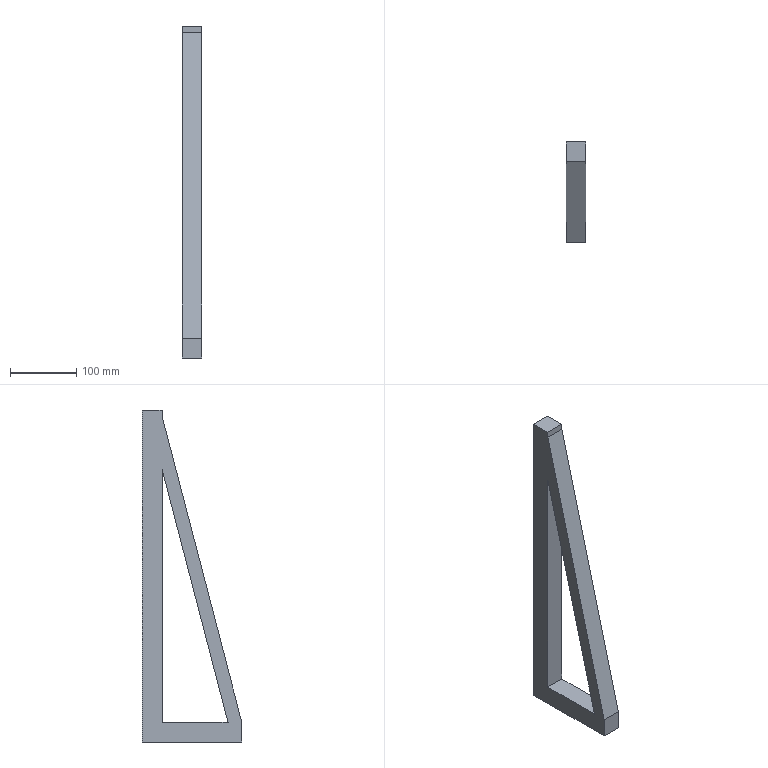Component | SolidWorks | LiftingArm122-1 | 1 solid | 11 faces | box 30 x 150 x 500 mm | volume 818896 mm3 | plane 11
build123d program:
from build123d import *

# Parameters (mm, degrees)
BOSS_EXTRUDE1_DEPTH = 30


with BuildPart() as part:
    # Sketch1 → Boss-Extrude1 (new body)
    with BuildSketch(Plane.XY):
        Polygon((0, 0), (500, 0), (500, -30), (490.421, -30), (30, -150), (0, -150), align=None)
        Polygon((30, -30), (411.12, -30), (30, -129.332), align=None, mode=Mode.SUBTRACT)
    extrude(amount=BOSS_EXTRUDE1_DEPTH)


solid = part.part

# Placed as in the assembly
solid = solid.moved(Location((-219.479, 25.652, 889.07), (0, -90, 0)))
STEP:
#1=COLOUR_RGB('',0.7922,0.8196,0.9333);
#2=FILL_AREA_STYLE_COLOUR('',#1);
#3=FILL_AREA_STYLE('',(#2));
#4=SURFACE_STYLE_FILL_AREA(#3);
#5=SURFACE_SIDE_STYLE('',(#4));
#6=SURFACE_STYLE_USAGE(.BOTH.,#5);
#7=PRESENTATION_STYLE_ASSIGNMENT((#6));
#8=CARTESIAN_POINT('',(-9.822,1.01,35.003));
#9=VERTEX_POINT('',#8);
#10=CARTESIAN_POINT('',(-9.822,-4.896,35.003));
#11=VERTEX_POINT('',#10);
#12=CARTESIAN_POINT('',(-9.822,-4.896,35.003));
#13=DIRECTION('',(0.,-1.,0.));
#14=VECTOR('',#13,39.37);
#15=LINE('',#12,#14);
#16=EDGE_CURVE('',#9,#11,#15,.T.);
#17=ORIENTED_EDGE('',*,*,#16,.T.);
#18=CARTESIAN_POINT('',(-9.822,-4.896,36.184));
#19=VERTEX_POINT('',#18);
#20=CARTESIAN_POINT('',(-9.822,-4.896,36.184));
#21=DIRECTION('',(0.,0.,1.));
#22=VECTOR('',#21,39.37);
#23=LINE('',#20,#22);
#24=EDGE_CURVE('',#11,#19,#23,.T.);
#25=ORIENTED_EDGE('',*,*,#24,.T.);
#26=CARTESIAN_POINT('',(-9.822,-0.1712,54.311));
#27=VERTEX_POINT('',#26);
#28=CARTESIAN_POINT('',(-9.822,-4.896,36.184));
#29=DIRECTION('',(0.,0.2522,0.9677));
#30=VECTOR('',#29,39.37);
#31=LINE('',#28,#30);
#32=EDGE_CURVE('',#19,#27,#31,.T.);
#33=ORIENTED_EDGE('',*,*,#32,.T.);
#34=CARTESIAN_POINT('',(-9.822,-0.1712,54.688));
#35=VERTEX_POINT('',#34);
#36=CARTESIAN_POINT('',(-9.822,-0.1712,54.311));
#37=DIRECTION('',(0.,0.,1.));
#38=VECTOR('',#37,39.37);
#39=LINE('',#36,#38);
#40=EDGE_CURVE('',#27,#35,#39,.T.);
#41=ORIENTED_EDGE('',*,*,#40,.T.);
#42=CARTESIAN_POINT('',(-9.822,1.01,54.688));
#43=VERTEX_POINT('',#42);
#44=CARTESIAN_POINT('',(-9.822,1.01,54.688));
#45=DIRECTION('',(0.,1.,0.));
#46=VECTOR('',#45,39.37);
#47=LINE('',#44,#46);
#48=EDGE_CURVE('',#35,#43,#47,.T.);
#49=ORIENTED_EDGE('',*,*,#48,.T.);
#50=CARTESIAN_POINT('',(-9.822,1.01,35.003));
#51=DIRECTION('',(0.,0.,-1.));
#52=VECTOR('',#51,39.37);
#53=LINE('',#50,#52);
#54=EDGE_CURVE('',#43,#9,#53,.T.);
#55=ORIENTED_EDGE('',*,*,#54,.T.);
#56=EDGE_LOOP('',(#17,#25,#33,#41,#49,#55));
#57=FACE_OUTER_BOUND('',#56,.T.);
#58=CARTESIAN_POINT('',(-9.822,-4.082,36.184));
#59=VERTEX_POINT('',#58);
#60=CARTESIAN_POINT('',(-9.822,-0.1712,51.189));
#61=VERTEX_POINT('',#60);
#62=CARTESIAN_POINT('',(-9.822,-4.082,36.184));
#63=DIRECTION('',(0.,0.2522,0.9677));
#64=VECTOR('',#63,39.37);
#65=LINE('',#62,#64);
#66=EDGE_CURVE('',#59,#61,#65,.T.);
#67=ORIENTED_EDGE('',*,*,#66,.F.);
#68=CARTESIAN_POINT('',(-9.822,-0.1712,36.184));
#69=VERTEX_POINT('',#68);
#70=CARTESIAN_POINT('',(-9.822,-0.1712,36.184));
#71=DIRECTION('',(0.,-1.,0.));
#72=VECTOR('',#71,39.37);
#73=LINE('',#70,#72);
#74=EDGE_CURVE('',#69,#59,#73,.T.);
#75=ORIENTED_EDGE('',*,*,#74,.F.);
#76=CARTESIAN_POINT('',(-9.822,-0.1712,36.184));
#77=DIRECTION('',(0.,-0.,-1.));
#78=VECTOR('',#77,39.37);
#79=LINE('',#76,#78);
#80=EDGE_CURVE('',#61,#69,#79,.T.);
#81=ORIENTED_EDGE('',*,*,#80,.F.);
#82=EDGE_LOOP('',(#67,#75,#81));
#83=FACE_BOUND('',#82,.T.);
#84=CARTESIAN_POINT('',(-9.822,1.01,35.003));
#85=DIRECTION('',(1.,0.,0.));
#86=DIRECTION('',(0.,0.,-1.));
#87=AXIS2_PLACEMENT_3D('',#84,#85,#86);
#88=PLANE('',#87);
#89=ADVANCED_FACE('',(#57,#83),#88,.F.);
#90=CARTESIAN_POINT('',(-8.641,1.01,35.003));
#91=VERTEX_POINT('',#90);
#92=CARTESIAN_POINT('',(-8.641,-4.896,35.003));
#93=VERTEX_POINT('',#92);
#94=CARTESIAN_POINT('',(-8.641,-4.896,35.003));
#95=DIRECTION('',(0.,-1.,0.));
#96=VECTOR('',#95,39.37);
#97=LINE('',#94,#96);
#98=EDGE_CURVE('',#91,#93,#97,.T.);
#99=ORIENTED_EDGE('',*,*,#98,.F.);
#100=CARTESIAN_POINT('',(-8.641,1.01,54.688));
#101=VERTEX_POINT('',#100);
#102=CARTESIAN_POINT('',(-8.641,1.01,35.003));
#103=DIRECTION('',(0.,0.,-1.));
#104=VECTOR('',#103,39.37);
#105=LINE('',#102,#104);
#106=EDGE_CURVE('',#101,#91,#105,.T.);
#107=ORIENTED_EDGE('',*,*,#106,.F.);
#108=CARTESIAN_POINT('',(-8.641,-0.1712,54.688));
#109=VERTEX_POINT('',#108);
#110=CARTESIAN_POINT('',(-8.641,1.01,54.688));
#111=DIRECTION('',(0.,1.,0.));
#112=VECTOR('',#111,39.37);
#113=LINE('',#110,#112);
#114=EDGE_CURVE('',#109,#101,#113,.T.);
#115=ORIENTED_EDGE('',*,*,#114,.F.);
#116=CARTESIAN_POINT('',(-8.641,-0.1712,54.311));
#117=VERTEX_POINT('',#116);
#118=CARTESIAN_POINT('',(-8.641,-0.1712,54.311));
#119=DIRECTION('',(0.,0.,1.));
#120=VECTOR('',#119,39.37);
#121=LINE('',#118,#120);
#122=EDGE_CURVE('',#117,#109,#121,.T.);
#123=ORIENTED_EDGE('',*,*,#122,.F.);
#124=CARTESIAN_POINT('',(-8.641,-4.896,36.184));
#125=VERTEX_POINT('',#124);
#126=CARTESIAN_POINT('',(-8.641,-4.896,36.184));
#127=DIRECTION('',(0.,0.2522,0.9677));
#128=VECTOR('',#127,39.37);
#129=LINE('',#126,#128);
#130=EDGE_CURVE('',#125,#117,#129,.T.);
#131=ORIENTED_EDGE('',*,*,#130,.F.);
#132=CARTESIAN_POINT('',(-8.641,-4.896,36.184));
#133=DIRECTION('',(0.,0.,1.));
#134=VECTOR('',#133,39.37);
#135=LINE('',#132,#134);
#136=EDGE_CURVE('',#93,#125,#135,.T.);
#137=ORIENTED_EDGE('',*,*,#136,.F.);
#138=EDGE_LOOP('',(#99,#107,#115,#123,#131,#137));
#139=FACE_OUTER_BOUND('',#138,.T.);
#140=CARTESIAN_POINT('',(-8.641,-0.1712,36.184));
#141=VERTEX_POINT('',#140);
#142=CARTESIAN_POINT('',(-8.641,-4.082,36.184));
#143=VERTEX_POINT('',#142);
#144=CARTESIAN_POINT('',(-8.641,-0.1712,36.184));
#145=DIRECTION('',(0.,-1.,0.));
#146=VECTOR('',#145,39.37);
#147=LINE('',#144,#146);
#148=EDGE_CURVE('',#141,#143,#147,.T.);
#149=ORIENTED_EDGE('',*,*,#148,.T.);
#150=CARTESIAN_POINT('',(-8.641,-0.1712,51.189));
#151=VERTEX_POINT('',#150);
#152=CARTESIAN_POINT('',(-8.641,-4.082,36.184));
#153=DIRECTION('',(0.,0.2522,0.9677));
#154=VECTOR('',#153,39.37);
#155=LINE('',#152,#154);
#156=EDGE_CURVE('',#143,#151,#155,.T.);
#157=ORIENTED_EDGE('',*,*,#156,.T.);
#158=CARTESIAN_POINT('',(-8.641,-0.1712,36.184));
#159=DIRECTION('',(0.,-0.,-1.));
#160=VECTOR('',#159,39.37);
#161=LINE('',#158,#160);
#162=EDGE_CURVE('',#151,#141,#161,.T.);
#163=ORIENTED_EDGE('',*,*,#162,.T.);
#164=EDGE_LOOP('',(#149,#157,#163));
#165=FACE_BOUND('',#164,.T.);
#166=CARTESIAN_POINT('',(-8.641,1.01,35.003));
#167=DIRECTION('',(1.,0.,0.));
#168=DIRECTION('',(0.,0.,-1.));
#169=AXIS2_PLACEMENT_3D('',#166,#167,#168);
#170=PLANE('',#169);
#171=ADVANCED_FACE('',(#139,#165),#170,.T.);
#172=ORIENTED_EDGE('',*,*,#98,.T.);
#173=CARTESIAN_POINT('',(-9.822,-4.896,35.003));
#174=DIRECTION('',(1.,0.,0.));
#175=VECTOR('',#174,39.37);
#176=LINE('',#173,#175);
#177=EDGE_CURVE('',#11,#93,#176,.T.);
#178=ORIENTED_EDGE('',*,*,#177,.F.);
#179=ORIENTED_EDGE('',*,*,#16,.F.);
#180=CARTESIAN_POINT('',(-9.822,1.01,35.003));
#181=DIRECTION('',(1.,0.,0.));
#182=VECTOR('',#181,39.37);
#183=LINE('',#180,#182);
#184=EDGE_CURVE('',#9,#91,#183,.T.);
#185=ORIENTED_EDGE('',*,*,#184,.T.);
#186=EDGE_LOOP('',(#172,#178,#179,#185));
#187=FACE_OUTER_BOUND('',#186,.T.);
#188=CARTESIAN_POINT('',(-9.822,-4.896,35.003));
#189=DIRECTION('',(0.,0.,1.));
#190=DIRECTION('',(1.,0.,0.));
#191=AXIS2_PLACEMENT_3D('',#188,#189,#190);
#192=PLANE('',#191);
#193=ADVANCED_FACE('',(#187),#192,.F.);
#194=ORIENTED_EDGE('',*,*,#136,.T.);
#195=CARTESIAN_POINT('',(-9.822,-4.896,36.184));
#196=DIRECTION('',(1.,0.,0.));
#197=VECTOR('',#196,39.37);
#198=LINE('',#195,#197);
#199=EDGE_CURVE('',#19,#125,#198,.T.);
#200=ORIENTED_EDGE('',*,*,#199,.F.);
#201=ORIENTED_EDGE('',*,*,#24,.F.);
#202=ORIENTED_EDGE('',*,*,#177,.T.);
#203=EDGE_LOOP('',(#194,#200,#201,#202));
#204=FACE_OUTER_BOUND('',#203,.T.);
#205=CARTESIAN_POINT('',(-9.822,-4.896,36.184));
#206=DIRECTION('',(0.,1.,0.));
#207=DIRECTION('',(-1.,0.,0.));
#208=AXIS2_PLACEMENT_3D('',#205,#206,#207);
#209=PLANE('',#208);
#210=ADVANCED_FACE('',(#204),#209,.F.);
#211=ORIENTED_EDGE('',*,*,#130,.T.);
#212=CARTESIAN_POINT('',(-9.822,-0.1712,54.311));
#213=DIRECTION('',(1.,0.,0.));
#214=VECTOR('',#213,39.37);
#215=LINE('',#212,#214);
#216=EDGE_CURVE('',#27,#117,#215,.T.);
#217=ORIENTED_EDGE('',*,*,#216,.F.);
#218=ORIENTED_EDGE('',*,*,#32,.F.);
#219=ORIENTED_EDGE('',*,*,#199,.T.);
#220=EDGE_LOOP('',(#211,#217,#218,#219));
#221=FACE_OUTER_BOUND('',#220,.T.);
#222=CARTESIAN_POINT('',(-9.822,-4.896,36.184));
#223=DIRECTION('',(0.,0.9677,-0.2522));
#224=DIRECTION('',(0.,-0.2522,-0.9677));
#225=AXIS2_PLACEMENT_3D('',#222,#223,#224);
#226=PLANE('',#225);
#227=ADVANCED_FACE('',(#221),#226,.F.);
#228=ORIENTED_EDGE('',*,*,#122,.T.);
#229=CARTESIAN_POINT('',(-9.822,-0.1712,54.688));
#230=DIRECTION('',(1.,0.,0.));
#231=VECTOR('',#230,39.37);
#232=LINE('',#229,#231);
#233=EDGE_CURVE('',#35,#109,#232,.T.);
#234=ORIENTED_EDGE('',*,*,#233,.F.);
#235=ORIENTED_EDGE('',*,*,#40,.F.);
#236=ORIENTED_EDGE('',*,*,#216,.T.);
#237=EDGE_LOOP('',(#228,#234,#235,#236));
#238=FACE_OUTER_BOUND('',#237,.T.);
#239=CARTESIAN_POINT('',(-9.822,-0.1712,54.311));
#240=DIRECTION('',(0.,1.,0.));
#241=DIRECTION('',(-1.,0.,0.));
#242=AXIS2_PLACEMENT_3D('',#239,#240,#241);
#243=PLANE('',#242);
#244=ADVANCED_FACE('',(#238),#243,.F.);
#245=ORIENTED_EDGE('',*,*,#114,.T.);
#246=CARTESIAN_POINT('',(-9.822,1.01,54.688));
#247=DIRECTION('',(1.,0.,0.));
#248=VECTOR('',#247,39.37);
#249=LINE('',#246,#248);
#250=EDGE_CURVE('',#43,#101,#249,.T.);
#251=ORIENTED_EDGE('',*,*,#250,.F.);
#252=ORIENTED_EDGE('',*,*,#48,.F.);
#253=ORIENTED_EDGE('',*,*,#233,.T.);
#254=EDGE_LOOP('',(#245,#251,#252,#253));
#255=FACE_OUTER_BOUND('',#254,.T.);
#256=CARTESIAN_POINT('',(-9.822,1.01,54.688));
#257=DIRECTION('',(0.,0.,-1.));
#258=DIRECTION('',(-1.,0.,0.));
#259=AXIS2_PLACEMENT_3D('',#256,#257,#258);
#260=PLANE('',#259);
#261=ADVANCED_FACE('',(#255),#260,.F.);
#262=ORIENTED_EDGE('',*,*,#106,.T.);
#263=ORIENTED_EDGE('',*,*,#184,.F.);
#264=ORIENTED_EDGE('',*,*,#54,.F.);
#265=ORIENTED_EDGE('',*,*,#250,.T.);
#266=EDGE_LOOP('',(#262,#263,#264,#265));
#267=FACE_OUTER_BOUND('',#266,.T.);
#268=CARTESIAN_POINT('',(-9.822,1.01,35.003));
#269=DIRECTION('',(0.,-1.,0.));
#270=DIRECTION('',(1.,0.,0.));
#271=AXIS2_PLACEMENT_3D('',#268,#269,#270);
#272=PLANE('',#271);
#273=ADVANCED_FACE('',(#267),#272,.F.);
#274=ORIENTED_EDGE('',*,*,#156,.F.);
#275=CARTESIAN_POINT('',(-9.822,-4.082,36.184));
#276=DIRECTION('',(1.,0.,0.));
#277=VECTOR('',#276,39.37);
#278=LINE('',#275,#277);
#279=EDGE_CURVE('',#59,#143,#278,.T.);
#280=ORIENTED_EDGE('',*,*,#279,.F.);
#281=ORIENTED_EDGE('',*,*,#66,.T.);
#282=CARTESIAN_POINT('',(-9.822,-0.1712,51.189));
#283=DIRECTION('',(1.,0.,0.));
#284=VECTOR('',#283,39.37);
#285=LINE('',#282,#284);
#286=EDGE_CURVE('',#61,#151,#285,.T.);
#287=ORIENTED_EDGE('',*,*,#286,.T.);
#288=EDGE_LOOP('',(#274,#280,#281,#287));
#289=FACE_OUTER_BOUND('',#288,.T.);
#290=CARTESIAN_POINT('',(-9.822,-4.082,36.184));
#291=DIRECTION('',(0.,0.9677,-0.2522));
#292=DIRECTION('',(0.,-0.2522,-0.9677));
#293=AXIS2_PLACEMENT_3D('',#290,#291,#292);
#294=PLANE('',#293);
#295=ADVANCED_FACE('',(#289),#294,.T.);
#296=ORIENTED_EDGE('',*,*,#162,.F.);
#297=ORIENTED_EDGE('',*,*,#286,.F.);
#298=ORIENTED_EDGE('',*,*,#80,.T.);
#299=CARTESIAN_POINT('',(-9.822,-0.1712,36.184));
#300=DIRECTION('',(1.,0.,0.));
#301=VECTOR('',#300,39.37);
#302=LINE('',#299,#301);
#303=EDGE_CURVE('',#69,#141,#302,.T.);
#304=ORIENTED_EDGE('',*,*,#303,.T.);
#305=EDGE_LOOP('',(#296,#297,#298,#304));
#306=FACE_OUTER_BOUND('',#305,.T.);
#307=CARTESIAN_POINT('',(-9.822,-0.1712,36.184));
#308=DIRECTION('',(0.,-1.,0.));
#309=DIRECTION('',(0.,0.,1.));
#310=AXIS2_PLACEMENT_3D('',#307,#308,#309);
#311=PLANE('',#310);
#312=ADVANCED_FACE('',(#306),#311,.T.);
#313=ORIENTED_EDGE('',*,*,#148,.F.);
#314=ORIENTED_EDGE('',*,*,#303,.F.);
#315=ORIENTED_EDGE('',*,*,#74,.T.);
#316=ORIENTED_EDGE('',*,*,#279,.T.);
#317=EDGE_LOOP('',(#313,#314,#315,#316));
#318=FACE_OUTER_BOUND('',#317,.T.);
#319=CARTESIAN_POINT('',(-9.822,-0.1712,36.184));
#320=DIRECTION('',(0.,0.,1.));
#321=DIRECTION('',(0.,1.,-0.));
#322=AXIS2_PLACEMENT_3D('',#319,#320,#321);
#323=PLANE('',#322);
#324=ADVANCED_FACE('',(#318),#323,.T.);
#325=CLOSED_SHELL('',(#89,#171,#193,#210,#227,#244,#261,#273,#295,#312,#324));
#326=MANIFOLD_SOLID_BREP('',#325);
#327=STYLED_ITEM('',(#7),#326);
#328=PRESENTATION_LAYER_ASSIGNMENT('','',(#327));
#329=CARTESIAN_POINT('',(0.,0.,0.));
#330=DIRECTION('',(0.,0.,1.));
#331=DIRECTION('',(1.,0.,0.));
#332=AXIS2_PLACEMENT_3D('',#329,#330,#331);
#333=(LENGTH_UNIT()NAMED_UNIT(*)SI_UNIT($,.METRE.));
#334=LENGTH_MEASURE_WITH_UNIT(LENGTH_MEASURE(0.0254),#333);
#335=DIMENSIONAL_EXPONENTS(1.,0.,0.,0.,0.,0.,0.);
#336=(CONVERSION_BASED_UNIT('',#334)LENGTH_UNIT()NAMED_UNIT(#335));
#337=UNCERTAINTY_MEASURE_WITH_UNIT(LENGTH_MEASURE(0.00001),#336,'','');
#338=(NAMED_UNIT(*)PLANE_ANGLE_UNIT()SI_UNIT($,.RADIAN.));
#339=(NAMED_UNIT(*)SI_UNIT($,.STERADIAN.)SOLID_ANGLE_UNIT());
#340=(GEOMETRIC_REPRESENTATION_CONTEXT(3)GLOBAL_UNCERTAINTY_ASSIGNED_CONTEXT((#337))GLOBAL_UNIT_ASSIGNED_CONTEXT((#336,#338,#339))REPRESENTATION_CONTEXT('',''));
#341=ADVANCED_BREP_SHAPE_REPRESENTATION('',(#326,#332),#340);
#342=(LENGTH_UNIT()NAMED_UNIT(*)SI_UNIT($,.METRE.));
#343=LENGTH_MEASURE_WITH_UNIT(LENGTH_MEASURE(0.0254),#342);
#344=DIMENSIONAL_EXPONENTS(1.,0.,0.,0.,0.,0.,0.);
#345=(CONVERSION_BASED_UNIT('',#343)LENGTH_UNIT()NAMED_UNIT(#344));
#346=UNCERTAINTY_MEASURE_WITH_UNIT(LENGTH_MEASURE(0.00001),#345,'','');
#347=(NAMED_UNIT(*)PLANE_ANGLE_UNIT()SI_UNIT($,.RADIAN.));
#348=(NAMED_UNIT(*)SI_UNIT($,.STERADIAN.)SOLID_ANGLE_UNIT());
#349=(GEOMETRIC_REPRESENTATION_CONTEXT(3)GLOBAL_UNCERTAINTY_ASSIGNED_CONTEXT((#346))GLOBAL_UNIT_ASSIGNED_CONTEXT((#345,#347,#348))REPRESENTATION_CONTEXT('',''));
#350=MECHANICAL_DESIGN_GEOMETRIC_PRESENTATION_REPRESENTATION('',(#327),#349);